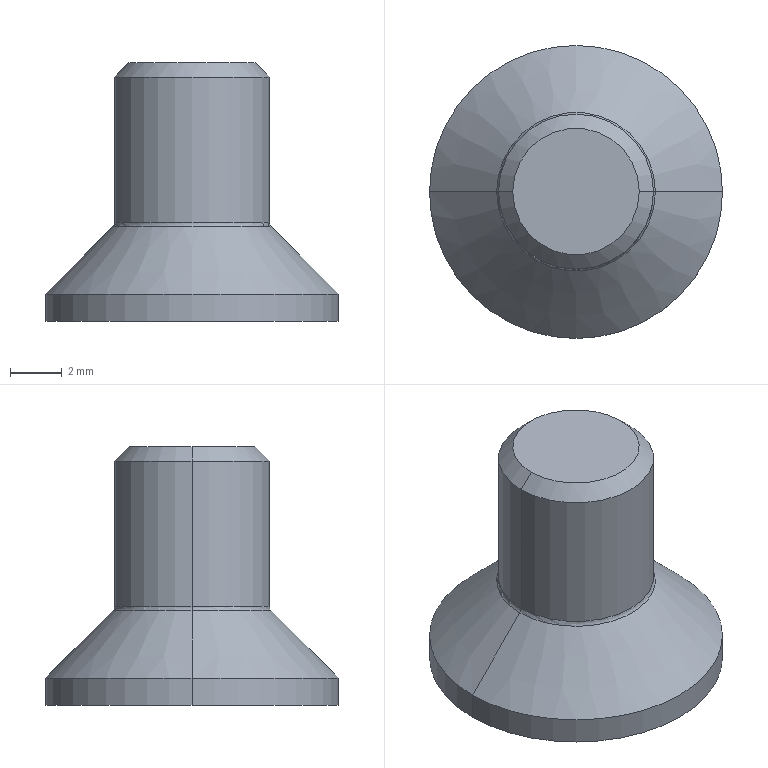Component | SolidWorks | hexagon socket countersunk head screws gb-1 | 1 solid | 26 faces | box 11.34 x 11.34 x 10 mm | volume 423 mm3 | plane 14 | cone 6 | cylinder 4 | torus 2 | commonest cylinder face diameters 11.34 x2 6 x2
build123d program:
from build123d import *

# Parameters (mm, degrees)
HEXAGONSOCKET_DEPTH = 1.1
HEADFILLET_R        = 0.25
CHAMFER_2_SIZE      = 0.55
SKETCH4_W           = 5
SKETCH4_H           = 5


with BuildPart() as part:
    # Sketch1 → Base (revolve)
    with BuildSketch(Plane.XY, mode=Mode.PRIVATE) as base_sk:
        Polygon((0, 0), (0, 6.72), (3.72, 3), (10, 3), (10, 0), align=None)
    revolve(base_sk.sketch.rotate(Axis((-0.5871, 0, 0), (1, 0, 0)), 90), axis=Axis((-0.5871, 0, 0), (1, 0, 0)))

    # Sketch2 → HexagonSocket (cut)
    with BuildSketch(Plane(origin=(0, 0, 0), x_dir=(0, 0, -1), z_dir=(1, 0, 0))):
        Polygon((2.309, 0), (1.155, 2), (-1.155, 2), (-2.309, 0), (-1.155, -2), (1.155, -2), align=None)
    extrude(amount=HEXAGONSOCKET_DEPTH, mode=Mode.SUBTRACT)

    # Sketch3 → Cut-Revolve1 (revolve, cut)
    with BuildSketch(Plane.XY, mode=Mode.PRIVATE) as cut_revolve1_sk:
        Polygon((1.1, 2), (2.255, 0), (1.1, 0), align=None)
    revolve(cut_revolve1_sk.sketch.rotate(Axis((-0.4391, 0, 0), (1, 0, 0)), 90), axis=Axis((-0.4391, 0, 0), (1, 0, 0)), mode=Mode.SUBTRACT)

    # HeadFillet
    headfillet_edges = [part.edges().sort_by_distance(p)[0] for p in [
        (3.72, 0, -3),
    ]]
    fillet(headfillet_edges, radius=HEADFILLET_R)

    # Chamfer 2
    chamfer_2_edges = [part.edges().sort_by_distance(p)[0] for p in [
        (10, 0, -3),
    ]]
    chamfer(chamfer_2_edges, length=CHAMFER_2_SIZE)

    # Sketch4 → Cut-Revolve2 (revolve, cut)
    with BuildSketch(Plane(origin=(0, 0, 0), x_dir=(1, 0, 0), z_dir=(0, 1, 0)), mode=Mode.PRIVATE) as cut_revolve2_sk:
        with Locations((0.5, 8.17)):
            Rectangle(SKETCH4_W, SKETCH4_H)
    revolve(cut_revolve2_sk.sketch.rotate(Axis((11.853, 0, 0), (-1, 0, 0)), 180), axis=Axis((11.853, 0, 0), (-1, 0, 0)), mode=Mode.SUBTRACT)


solid = part.part

# Placed as in the assembly
solid = solid.moved(Location((21.481, 88.385, 42.5), (0, -90, 0)))
STEP:
#1=CARTESIAN_POINT('',(0.8457,3.48,1.762));
#2=VERTEX_POINT('',#1);
#3=CARTESIAN_POINT('',(0.767,3.48,1.717));
#4=VERTEX_POINT('',#3);
#5=CARTESIAN_POINT('',(0.8457,3.48,1.762));
#6=DIRECTION('',(-0.866,-0.,-0.5));
#7=VECTOR('',#6,39.37);
#8=LINE('',#5,#7);
#9=EDGE_CURVE('',#2,#4,#8,.T.);
#10=ORIENTED_EDGE('',*,*,#9,.F.);
#11=CARTESIAN_POINT('',(0.9244,3.48,1.717));
#12=VERTEX_POINT('',#11);
#13=CARTESIAN_POINT('',(0.8457,3.48,1.762));
#14=DIRECTION('',(0.866,0.,-0.5));
#15=VECTOR('',#14,39.37);
#16=LINE('',#13,#15);
#17=EDGE_CURVE('',#2,#12,#16,.T.);
#18=ORIENTED_EDGE('',*,*,#17,.T.);
#19=CARTESIAN_POINT('',(0.9139,3.44,1.717));
#20=VERTEX_POINT('',#19);
#21=CARTESIAN_POINT('',(0.8457,3.48,1.717));
#22=DIRECTION('',(0.,-0.,-1.));
#23=DIRECTION('',(-1.,0.,0.));
#24=AXIS2_PLACEMENT_3D('',#21,#22,#23);
#25=CIRCLE('',#24,0.07874);
#26=EDGE_CURVE('',#12,#20,#25,.T.);
#27=ORIENTED_EDGE('',*,*,#26,.T.);
#28=CARTESIAN_POINT('',(0.8457,3.401,1.717));
#29=VERTEX_POINT('',#28);
#30=CARTESIAN_POINT('',(0.8457,3.48,1.717));
#31=DIRECTION('',(0.,-0.,-1.));
#32=DIRECTION('',(-1.,0.,0.));
#33=AXIS2_PLACEMENT_3D('',#30,#31,#32);
#34=CIRCLE('',#33,0.07874);
#35=EDGE_CURVE('',#20,#29,#34,.T.);
#36=ORIENTED_EDGE('',*,*,#35,.T.);
#37=CARTESIAN_POINT('',(0.7775,3.44,1.717));
#38=VERTEX_POINT('',#37);
#39=CARTESIAN_POINT('',(0.8457,3.48,1.717));
#40=DIRECTION('',(0.,-0.,-1.));
#41=DIRECTION('',(-1.,0.,0.));
#42=AXIS2_PLACEMENT_3D('',#39,#40,#41);
#43=CIRCLE('',#42,0.07874);
#44=EDGE_CURVE('',#29,#38,#43,.T.);
#45=ORIENTED_EDGE('',*,*,#44,.T.);
#46=CARTESIAN_POINT('',(0.8457,3.48,1.717));
#47=DIRECTION('',(0.,-0.,-1.));
#48=DIRECTION('',(-1.,0.,0.));
#49=AXIS2_PLACEMENT_3D('',#46,#47,#48);
#50=CIRCLE('',#49,0.07874);
#51=EDGE_CURVE('',#38,#4,#50,.T.);
#52=ORIENTED_EDGE('',*,*,#51,.T.);
#53=EDGE_LOOP('',(#10,#18,#27,#36,#45,#52));
#54=FACE_OUTER_BOUND('',#53,.T.);
#55=CARTESIAN_POINT('',(0.8457,3.48,-37.608));
#56=DIRECTION('',(0.,-0.,-1.));
#57=DIRECTION('',(-1.,-0.,0.));
#58=AXIS2_PLACEMENT_3D('',#55,#56,#57);
#59=CONICAL_SURFACE('',#58,68.191,1.047);
#60=ADVANCED_FACE('',(#54),#59,.F.);
#61=CARTESIAN_POINT('',(0.6225,3.48,1.673));
#62=VERTEX_POINT('',#61);
#63=CARTESIAN_POINT('',(1.069,3.48,1.673));
#64=VERTEX_POINT('',#63);
#65=CARTESIAN_POINT('',(0.8457,3.48,1.673));
#66=DIRECTION('',(0.,-0.,-1.));
#67=DIRECTION('',(1.,0.,0.));
#68=AXIS2_PLACEMENT_3D('',#65,#66,#67);
#69=CIRCLE('',#68,0.2232);
#70=EDGE_CURVE('',#62,#64,#69,.T.);
#71=ORIENTED_EDGE('',*,*,#70,.F.);
#72=CARTESIAN_POINT('',(0.6225,3.48,1.715));
#73=VERTEX_POINT('',#72);
#74=CARTESIAN_POINT('',(0.6225,3.48,2.14));
#75=DIRECTION('',(-0.,0.,1.));
#76=VECTOR('',#75,39.37);
#77=LINE('',#74,#76);
#78=EDGE_CURVE('',#62,#73,#77,.T.);
#79=ORIENTED_EDGE('',*,*,#78,.T.);
#80=CARTESIAN_POINT('',(1.069,3.48,1.715));
#81=VERTEX_POINT('',#80);
#82=CARTESIAN_POINT('',(0.8457,3.48,1.715));
#83=DIRECTION('',(-0.,0.,1.));
#84=DIRECTION('',(-1.,0.,0.));
#85=AXIS2_PLACEMENT_3D('',#82,#83,#84);
#86=CIRCLE('',#85,0.2232);
#87=EDGE_CURVE('',#81,#73,#86,.T.);
#88=ORIENTED_EDGE('',*,*,#87,.F.);
#89=CARTESIAN_POINT('',(1.069,3.48,2.14));
#90=DIRECTION('',(-0.,0.,1.));
#91=VECTOR('',#90,39.37);
#92=LINE('',#89,#91);
#93=EDGE_CURVE('',#64,#81,#92,.T.);
#94=ORIENTED_EDGE('',*,*,#93,.F.);
#95=EDGE_LOOP('',(#71,#79,#88,#94));
#96=FACE_OUTER_BOUND('',#95,.T.);
#97=CARTESIAN_POINT('',(0.8457,3.48,2.14));
#98=DIRECTION('',(-0.,0.,1.));
#99=DIRECTION('',(1.,0.,0.));
#100=AXIS2_PLACEMENT_3D('',#97,#98,#99);
#101=CYLINDRICAL_SURFACE('',#100,0.2232);
#102=ADVANCED_FACE('',(#96),#101,.T.);
#103=CARTESIAN_POINT('',(0.9422,3.48,2.067));
#104=VERTEX_POINT('',#103);
#105=CARTESIAN_POINT('',(0.7492,3.48,2.067));
#106=VERTEX_POINT('',#105);
#107=CARTESIAN_POINT('',(0.8457,3.48,2.067));
#108=DIRECTION('',(-0.,0.,1.));
#109=DIRECTION('',(-1.,0.,0.));
#110=AXIS2_PLACEMENT_3D('',#107,#108,#109);
#111=CIRCLE('',#110,0.09646);
#112=EDGE_CURVE('',#104,#106,#111,.T.);
#113=ORIENTED_EDGE('',*,*,#112,.F.);
#114=CARTESIAN_POINT('',(0.9638,3.48,2.045));
#115=VERTEX_POINT('',#114);
#116=CARTESIAN_POINT('',(0.9638,3.48,2.045));
#117=DIRECTION('',(0.7071,0.,-0.7071));
#118=VECTOR('',#117,39.37);
#119=LINE('',#116,#118);
#120=EDGE_CURVE('',#104,#115,#119,.T.);
#121=ORIENTED_EDGE('',*,*,#120,.T.);
#122=CARTESIAN_POINT('',(0.7276,3.48,2.045));
#123=VERTEX_POINT('',#122);
#124=CARTESIAN_POINT('',(0.8457,3.48,2.045));
#125=DIRECTION('',(0.,-0.,-1.));
#126=DIRECTION('',(-1.,0.,0.));
#127=AXIS2_PLACEMENT_3D('',#124,#125,#126);
#128=CIRCLE('',#127,0.1181);
#129=EDGE_CURVE('',#123,#115,#128,.T.);
#130=ORIENTED_EDGE('',*,*,#129,.F.);
#131=CARTESIAN_POINT('',(0.7276,3.48,2.045));
#132=DIRECTION('',(-0.7071,-0.,-0.7071));
#133=VECTOR('',#132,39.37);
#134=LINE('',#131,#133);
#135=EDGE_CURVE('',#106,#123,#134,.T.);
#136=ORIENTED_EDGE('',*,*,#135,.F.);
#137=EDGE_LOOP('',(#113,#121,#130,#136));
#138=FACE_OUTER_BOUND('',#137,.T.);
#139=CARTESIAN_POINT('',(0.8457,3.48,2.045));
#140=DIRECTION('',(0.,-0.,-1.));
#141=DIRECTION('',(-1.,0.,0.));
#142=AXIS2_PLACEMENT_3D('',#139,#140,#141);
#143=CONICAL_SURFACE('',#142,0.1181,0.7854);
#144=ADVANCED_FACE('',(#138),#143,.T.);
#145=CARTESIAN_POINT('',(0.9667,3.48,1.817));
#146=VERTEX_POINT('',#145);
#147=CARTESIAN_POINT('',(0.7247,3.48,1.817));
#148=VERTEX_POINT('',#147);
#149=CARTESIAN_POINT('',(0.8457,3.48,1.817));
#150=DIRECTION('',(0.,-0.,-1.));
#151=DIRECTION('',(-1.,0.,0.));
#152=AXIS2_PLACEMENT_3D('',#149,#150,#151);
#153=CIRCLE('',#152,0.121);
#154=EDGE_CURVE('',#146,#148,#153,.T.);
#155=ORIENTED_EDGE('',*,*,#154,.F.);
#156=CARTESIAN_POINT('',(0.9638,3.48,1.824));
#157=VERTEX_POINT('',#156);
#158=CARTESIAN_POINT('',(0.9736,3.48,1.824));
#159=DIRECTION('',(-0.,1.,-0.));
#160=DIRECTION('',(-1.,0.,0.));
#161=AXIS2_PLACEMENT_3D('',#158,#159,#160);
#162=CIRCLE('',#161,0.009843);
#163=EDGE_CURVE('',#146,#157,#162,.T.);
#164=ORIENTED_EDGE('',*,*,#163,.T.);
#165=CARTESIAN_POINT('',(0.7276,3.48,1.824));
#166=VERTEX_POINT('',#165);
#167=CARTESIAN_POINT('',(0.8457,3.48,1.824));
#168=DIRECTION('',(-0.,0.,1.));
#169=DIRECTION('',(-1.,0.,0.));
#170=AXIS2_PLACEMENT_3D('',#167,#168,#169);
#171=CIRCLE('',#170,0.1181);
#172=EDGE_CURVE('',#166,#157,#171,.T.);
#173=ORIENTED_EDGE('',*,*,#172,.F.);
#174=CARTESIAN_POINT('',(0.7177,3.48,1.824));
#175=DIRECTION('',(0.,-1.,0.));
#176=DIRECTION('',(0.,0.,-1.));
#177=AXIS2_PLACEMENT_3D('',#174,#175,#176);
#178=CIRCLE('',#177,0.009843);
#179=EDGE_CURVE('',#148,#166,#178,.T.);
#180=ORIENTED_EDGE('',*,*,#179,.F.);
#181=EDGE_LOOP('',(#155,#164,#173,#180));
#182=FACE_OUTER_BOUND('',#181,.T.);
#183=CARTESIAN_POINT('',(0.8457,3.48,1.824));
#184=DIRECTION('',(0.,-0.,-1.));
#185=DIRECTION('',(-1.,-0.,-0.));
#186=AXIS2_PLACEMENT_3D('',#183,#184,#185);
#187=TOROIDAL_SURFACE('',#186,0.128,0.009843);
#188=ADVANCED_FACE('',(#182),#187,.F.);
#189=CARTESIAN_POINT('',(0.8457,3.48,1.817));
#190=DIRECTION('',(0.,-0.,-1.));
#191=DIRECTION('',(-1.,0.,0.));
#192=AXIS2_PLACEMENT_3D('',#189,#190,#191);
#193=CIRCLE('',#192,0.121);
#194=EDGE_CURVE('',#148,#146,#193,.T.);
#195=ORIENTED_EDGE('',*,*,#194,.T.);
#196=CARTESIAN_POINT('',(0.9638,3.48,1.82));
#197=DIRECTION('',(0.7071,0.,-0.7071));
#198=VECTOR('',#197,39.37);
#199=LINE('',#196,#198);
#200=EDGE_CURVE('',#146,#81,#199,.T.);
#201=ORIENTED_EDGE('',*,*,#200,.T.);
#202=ORIENTED_EDGE('',*,*,#87,.T.);
#203=CARTESIAN_POINT('',(0.7276,3.48,1.82));
#204=DIRECTION('',(-0.7071,-0.,-0.7071));
#205=VECTOR('',#204,39.37);
#206=LINE('',#203,#205);
#207=EDGE_CURVE('',#148,#73,#206,.T.);
#208=ORIENTED_EDGE('',*,*,#207,.F.);
#209=EDGE_LOOP('',(#195,#201,#202,#208));
#210=FACE_OUTER_BOUND('',#209,.T.);
#211=CARTESIAN_POINT('',(0.8457,3.48,1.82));
#212=DIRECTION('',(0.,-0.,-1.));
#213=DIRECTION('',(-1.,0.,0.));
#214=AXIS2_PLACEMENT_3D('',#211,#212,#213);
#215=CONICAL_SURFACE('',#214,0.1181,0.7854);
#216=ADVANCED_FACE('',(#210),#215,.T.);
#217=ORIENTED_EDGE('',*,*,#129,.T.);
#218=CARTESIAN_POINT('',(0.9638,3.48,1.65));
#219=DIRECTION('',(0.,-0.,-1.));
#220=VECTOR('',#219,39.37);
#221=LINE('',#218,#220);
#222=EDGE_CURVE('',#115,#157,#221,.T.);
#223=ORIENTED_EDGE('',*,*,#222,.T.);
#224=CARTESIAN_POINT('',(0.8457,3.48,1.824));
#225=DIRECTION('',(-0.,0.,1.));
#226=DIRECTION('',(-1.,0.,0.));
#227=AXIS2_PLACEMENT_3D('',#224,#225,#226);
#228=CIRCLE('',#227,0.1181);
#229=EDGE_CURVE('',#157,#166,#228,.T.);
#230=ORIENTED_EDGE('',*,*,#229,.T.);
#231=CARTESIAN_POINT('',(0.7276,3.48,1.65));
#232=DIRECTION('',(0.,-0.,-1.));
#233=VECTOR('',#232,39.37);
#234=LINE('',#231,#233);
#235=EDGE_CURVE('',#123,#166,#234,.T.);
#236=ORIENTED_EDGE('',*,*,#235,.F.);
#237=EDGE_LOOP('',(#217,#223,#230,#236));
#238=FACE_OUTER_BOUND('',#237,.T.);
#239=CARTESIAN_POINT('',(0.8457,3.48,1.65));
#240=DIRECTION('',(0.,-0.,-1.));
#241=DIRECTION('',(-1.,0.,0.));
#242=AXIS2_PLACEMENT_3D('',#239,#240,#241);
#243=CYLINDRICAL_SURFACE('',#242,0.1181);
#244=ADVANCED_FACE('',(#238),#243,.T.);
#245=CARTESIAN_POINT('',(0.8457,3.48,2.067));
#246=DIRECTION('',(-0.,0.,1.));
#247=DIRECTION('',(-1.,0.,0.));
#248=AXIS2_PLACEMENT_3D('',#245,#246,#247);
#249=CIRCLE('',#248,0.09646);
#250=EDGE_CURVE('',#106,#104,#249,.T.);
#251=ORIENTED_EDGE('',*,*,#250,.T.);
#252=ORIENTED_EDGE('',*,*,#112,.T.);
#253=EDGE_LOOP('',(#251,#252));
#254=FACE_OUTER_BOUND('',#253,.T.);
#255=CARTESIAN_POINT('',(0.8457,3.598,2.067));
#256=DIRECTION('',(0.,-0.,-1.));
#257=DIRECTION('',(-1.,-0.,-0.));
#258=AXIS2_PLACEMENT_3D('',#255,#256,#257);
#259=PLANE('',#258);
#260=ADVANCED_FACE('',(#254),#259,.F.);
#261=ORIENTED_EDGE('',*,*,#222,.F.);
#262=CARTESIAN_POINT('',(0.8457,3.48,2.045));
#263=DIRECTION('',(0.,-0.,-1.));
#264=DIRECTION('',(-1.,0.,0.));
#265=AXIS2_PLACEMENT_3D('',#262,#263,#264);
#266=CIRCLE('',#265,0.1181);
#267=EDGE_CURVE('',#115,#123,#266,.T.);
#268=ORIENTED_EDGE('',*,*,#267,.T.);
#269=ORIENTED_EDGE('',*,*,#235,.T.);
#270=ORIENTED_EDGE('',*,*,#172,.T.);
#271=EDGE_LOOP('',(#261,#268,#269,#270));
#272=FACE_OUTER_BOUND('',#271,.T.);
#273=CARTESIAN_POINT('',(0.8457,3.48,1.65));
#274=DIRECTION('',(0.,-0.,-1.));
#275=DIRECTION('',(-1.,0.,0.));
#276=AXIS2_PLACEMENT_3D('',#273,#274,#275);
#277=CYLINDRICAL_SURFACE('',#276,0.1181);
#278=ADVANCED_FACE('',(#272),#277,.T.);
#279=ORIENTED_EDGE('',*,*,#200,.F.);
#280=ORIENTED_EDGE('',*,*,#154,.T.);
#281=ORIENTED_EDGE('',*,*,#207,.T.);
#282=CARTESIAN_POINT('',(0.8457,3.48,1.715));
#283=DIRECTION('',(-0.,0.,1.));
#284=DIRECTION('',(-1.,0.,0.));
#285=AXIS2_PLACEMENT_3D('',#282,#283,#284);
#286=CIRCLE('',#285,0.2232);
#287=EDGE_CURVE('',#73,#81,#286,.T.);
#288=ORIENTED_EDGE('',*,*,#287,.T.);
#289=EDGE_LOOP('',(#279,#280,#281,#288));
#290=FACE_OUTER_BOUND('',#289,.T.);
#291=CARTESIAN_POINT('',(0.8457,3.48,1.82));
#292=DIRECTION('',(0.,-0.,-1.));
#293=DIRECTION('',(-1.,0.,0.));
#294=AXIS2_PLACEMENT_3D('',#291,#292,#293);
#295=CONICAL_SURFACE('',#294,0.1181,0.7854);
#296=ADVANCED_FACE('',(#290),#295,.T.);
#297=ORIENTED_EDGE('',*,*,#163,.F.);
#298=ORIENTED_EDGE('',*,*,#194,.F.);
#299=ORIENTED_EDGE('',*,*,#179,.T.);
#300=ORIENTED_EDGE('',*,*,#229,.F.);
#301=EDGE_LOOP('',(#297,#298,#299,#300));
#302=FACE_OUTER_BOUND('',#301,.T.);
#303=CARTESIAN_POINT('',(0.8457,3.48,1.824));
#304=DIRECTION('',(0.,-0.,-1.));
#305=DIRECTION('',(-1.,-0.,-0.));
#306=AXIS2_PLACEMENT_3D('',#303,#304,#305);
#307=TOROIDAL_SURFACE('',#306,0.128,0.009843);
#308=ADVANCED_FACE('',(#302),#307,.F.);
#309=ORIENTED_EDGE('',*,*,#120,.F.);
#310=ORIENTED_EDGE('',*,*,#250,.F.);
#311=ORIENTED_EDGE('',*,*,#135,.T.);
#312=ORIENTED_EDGE('',*,*,#267,.F.);
#313=EDGE_LOOP('',(#309,#310,#311,#312));
#314=FACE_OUTER_BOUND('',#313,.T.);
#315=CARTESIAN_POINT('',(0.8457,3.48,2.045));
#316=DIRECTION('',(0.,-0.,-1.));
#317=DIRECTION('',(-1.,0.,0.));
#318=AXIS2_PLACEMENT_3D('',#315,#316,#317);
#319=CONICAL_SURFACE('',#318,0.1181,0.7854);
#320=ADVANCED_FACE('',(#314),#319,.T.);
#321=ORIENTED_EDGE('',*,*,#78,.F.);
#322=CARTESIAN_POINT('',(0.8457,3.48,1.673));
#323=DIRECTION('',(0.,-0.,-1.));
#324=DIRECTION('',(1.,0.,0.));
#325=AXIS2_PLACEMENT_3D('',#322,#323,#324);
#326=CIRCLE('',#325,0.2232);
#327=EDGE_CURVE('',#64,#62,#326,.T.);
#328=ORIENTED_EDGE('',*,*,#327,.F.);
#329=ORIENTED_EDGE('',*,*,#93,.T.);
#330=ORIENTED_EDGE('',*,*,#287,.F.);
#331=EDGE_LOOP('',(#321,#328,#329,#330));
#332=FACE_OUTER_BOUND('',#331,.T.);
#333=CARTESIAN_POINT('',(0.8457,3.48,2.14));
#334=DIRECTION('',(-0.,0.,1.));
#335=DIRECTION('',(1.,0.,0.));
#336=AXIS2_PLACEMENT_3D('',#333,#334,#335);
#337=CYLINDRICAL_SURFACE('',#336,0.2232);
#338=ADVANCED_FACE('',(#332),#337,.T.);
#339=ORIENTED_EDGE('',*,*,#17,.F.);
#340=ORIENTED_EDGE('',*,*,#9,.T.);
#341=CARTESIAN_POINT('',(0.7775,3.519,1.717));
#342=VERTEX_POINT('',#341);
#343=CARTESIAN_POINT('',(0.8457,3.48,1.717));
#344=DIRECTION('',(0.,-0.,-1.));
#345=DIRECTION('',(-1.,0.,0.));
#346=AXIS2_PLACEMENT_3D('',#343,#344,#345);
#347=CIRCLE('',#346,0.07874);
#348=EDGE_CURVE('',#4,#342,#347,.T.);
#349=ORIENTED_EDGE('',*,*,#348,.T.);
#350=CARTESIAN_POINT('',(0.8457,3.558,1.717));
#351=VERTEX_POINT('',#350);
#352=CARTESIAN_POINT('',(0.8457,3.48,1.717));
#353=DIRECTION('',(0.,-0.,-1.));
#354=DIRECTION('',(-1.,0.,0.));
#355=AXIS2_PLACEMENT_3D('',#352,#353,#354);
#356=CIRCLE('',#355,0.07874);
#357=EDGE_CURVE('',#342,#351,#356,.T.);
#358=ORIENTED_EDGE('',*,*,#357,.T.);
#359=CARTESIAN_POINT('',(0.9139,3.519,1.717));
#360=VERTEX_POINT('',#359);
#361=CARTESIAN_POINT('',(0.8457,3.48,1.717));
#362=DIRECTION('',(0.,-0.,-1.));
#363=DIRECTION('',(-1.,0.,0.));
#364=AXIS2_PLACEMENT_3D('',#361,#362,#363);
#365=CIRCLE('',#364,0.07874);
#366=EDGE_CURVE('',#351,#360,#365,.T.);
#367=ORIENTED_EDGE('',*,*,#366,.T.);
#368=CARTESIAN_POINT('',(0.8457,3.48,1.717));
#369=DIRECTION('',(0.,-0.,-1.));
#370=DIRECTION('',(-1.,0.,0.));
#371=AXIS2_PLACEMENT_3D('',#368,#369,#370);
#372=CIRCLE('',#371,0.07874);
#373=EDGE_CURVE('',#360,#12,#372,.T.);
#374=ORIENTED_EDGE('',*,*,#373,.T.);
#375=EDGE_LOOP('',(#339,#340,#349,#358,#367,#374));
#376=FACE_OUTER_BOUND('',#375,.T.);
#377=CARTESIAN_POINT('',(0.8457,3.48,-37.608));
#378=DIRECTION('',(0.,-0.,-1.));
#379=DIRECTION('',(-1.,-0.,0.));
#380=AXIS2_PLACEMENT_3D('',#377,#378,#379);
#381=CONICAL_SURFACE('',#380,68.191,1.047);
#382=ADVANCED_FACE('',(#376),#381,.F.);
#383=ORIENTED_EDGE('',*,*,#44,.F.);
#384=CARTESIAN_POINT('',(0.8002,3.401,1.717));
#385=VERTEX_POINT('',#384);
#386=CARTESIAN_POINT('',(0.8002,3.401,1.717));
#387=DIRECTION('',(1.,0.,0.));
#388=VECTOR('',#387,39.37);
#389=LINE('',#386,#388);
#390=EDGE_CURVE('',#385,#29,#389,.T.);
#391=ORIENTED_EDGE('',*,*,#390,.F.);
#392=CARTESIAN_POINT('',(0.7548,3.48,1.717));
#393=DIRECTION('',(0.5,-0.866,0.));
#394=VECTOR('',#393,39.37);
#395=LINE('',#392,#394);
#396=EDGE_CURVE('',#38,#385,#395,.T.);
#397=ORIENTED_EDGE('',*,*,#396,.F.);
#398=EDGE_LOOP('',(#383,#391,#397));
#399=FACE_OUTER_BOUND('',#398,.T.);
#400=CARTESIAN_POINT('',(0.9366,3.48,1.717));
#401=DIRECTION('',(-0.,0.,1.));
#402=DIRECTION('',(1.,0.,0.));
#403=AXIS2_PLACEMENT_3D('',#400,#401,#402);
#404=PLANE('',#403);
#405=ADVANCED_FACE('',(#399),#404,.F.);
#406=ORIENTED_EDGE('',*,*,#51,.F.);
#407=CARTESIAN_POINT('',(0.7548,3.48,1.717));
#408=VERTEX_POINT('',#407);
#409=CARTESIAN_POINT('',(0.7548,3.48,1.717));
#410=DIRECTION('',(0.5,-0.866,0.));
#411=VECTOR('',#410,39.37);
#412=LINE('',#409,#411);
#413=EDGE_CURVE('',#408,#38,#412,.T.);
#414=ORIENTED_EDGE('',*,*,#413,.F.);
#415=CARTESIAN_POINT('',(0.8002,3.558,1.717));
#416=DIRECTION('',(-0.5,-0.866,0.));
#417=VECTOR('',#416,39.37);
#418=LINE('',#415,#417);
#419=EDGE_CURVE('',#342,#408,#418,.T.);
#420=ORIENTED_EDGE('',*,*,#419,.F.);
#421=ORIENTED_EDGE('',*,*,#348,.F.);
#422=EDGE_LOOP('',(#406,#414,#420,#421));
#423=FACE_OUTER_BOUND('',#422,.T.);
#424=CARTESIAN_POINT('',(0.9366,3.48,1.717));
#425=DIRECTION('',(-0.,0.,1.));
#426=DIRECTION('',(1.,0.,0.));
#427=AXIS2_PLACEMENT_3D('',#424,#425,#426);
#428=PLANE('',#427);
#429=ADVANCED_FACE('',(#423),#428,.F.);
#430=ORIENTED_EDGE('',*,*,#357,.F.);
#431=CARTESIAN_POINT('',(0.8002,3.558,1.717));
#432=VERTEX_POINT('',#431);
#433=CARTESIAN_POINT('',(0.8002,3.558,1.717));
#434=DIRECTION('',(-0.5,-0.866,0.));
#435=VECTOR('',#434,39.37);
#436=LINE('',#433,#435);
#437=EDGE_CURVE('',#432,#342,#436,.T.);
#438=ORIENTED_EDGE('',*,*,#437,.F.);
#439=CARTESIAN_POINT('',(0.8912,3.558,1.717));
#440=DIRECTION('',(-1.,-0.,-0.));
#441=VECTOR('',#440,39.37);
#442=LINE('',#439,#441);
#443=EDGE_CURVE('',#351,#432,#442,.T.);
#444=ORIENTED_EDGE('',*,*,#443,.F.);
#445=EDGE_LOOP('',(#430,#438,#444));
#446=FACE_OUTER_BOUND('',#445,.T.);
#447=CARTESIAN_POINT('',(0.9366,3.48,1.717));
#448=DIRECTION('',(-0.,0.,1.));
#449=DIRECTION('',(1.,0.,0.));
#450=AXIS2_PLACEMENT_3D('',#447,#448,#449);
#451=PLANE('',#450);
#452=ADVANCED_FACE('',(#446),#451,.F.);
#453=ORIENTED_EDGE('',*,*,#366,.F.);
#454=CARTESIAN_POINT('',(0.8912,3.558,1.717));
#455=VERTEX_POINT('',#454);
#456=CARTESIAN_POINT('',(0.8912,3.558,1.717));
#457=DIRECTION('',(-1.,-0.,-0.));
#458=VECTOR('',#457,39.37);
#459=LINE('',#456,#458);
#460=EDGE_CURVE('',#455,#351,#459,.T.);
#461=ORIENTED_EDGE('',*,*,#460,.F.);
#462=CARTESIAN_POINT('',(0.9366,3.48,1.717));
#463=DIRECTION('',(-0.5,0.866,-0.));
#464=VECTOR('',#463,39.37);
#465=LINE('',#462,#464);
#466=EDGE_CURVE('',#360,#455,#465,.T.);
#467=ORIENTED_EDGE('',*,*,#466,.F.);
#468=EDGE_LOOP('',(#453,#461,#467));
#469=FACE_OUTER_BOUND('',#468,.T.);
#470=CARTESIAN_POINT('',(0.9366,3.48,1.717));
#471=DIRECTION('',(-0.,0.,1.));
#472=DIRECTION('',(1.,0.,0.));
#473=AXIS2_PLACEMENT_3D('',#470,#471,#472);
#474=PLANE('',#473);
#475=ADVANCED_FACE('',(#469),#474,.F.);
#476=ORIENTED_EDGE('',*,*,#373,.F.);
#477=CARTESIAN_POINT('',(0.9366,3.48,1.717));
#478=VERTEX_POINT('',#477);
#479=CARTESIAN_POINT('',(0.9366,3.48,1.717));
#480=DIRECTION('',(-0.5,0.866,-0.));
#481=VECTOR('',#480,39.37);
#482=LINE('',#479,#481);
#483=EDGE_CURVE('',#478,#360,#482,.T.);
#484=ORIENTED_EDGE('',*,*,#483,.F.);
#485=CARTESIAN_POINT('',(0.8912,3.401,1.717));
#486=DIRECTION('',(0.5,0.866,-0.));
#487=VECTOR('',#486,39.37);
#488=LINE('',#485,#487);
#489=EDGE_CURVE('',#20,#478,#488,.T.);
#490=ORIENTED_EDGE('',*,*,#489,.F.);
#491=ORIENTED_EDGE('',*,*,#26,.F.);
#492=EDGE_LOOP('',(#476,#484,#490,#491));
#493=FACE_OUTER_BOUND('',#492,.T.);
#494=CARTESIAN_POINT('',(0.9366,3.48,1.717));
#495=DIRECTION('',(-0.,0.,1.));
#496=DIRECTION('',(1.,0.,0.));
#497=AXIS2_PLACEMENT_3D('',#494,#495,#496);
#498=PLANE('',#497);
#499=ADVANCED_FACE('',(#493),#498,.F.);
#500=ORIENTED_EDGE('',*,*,#35,.F.);
#501=CARTESIAN_POINT('',(0.8912,3.401,1.717));
#502=VERTEX_POINT('',#501);
#503=CARTESIAN_POINT('',(0.8912,3.401,1.717));
#504=DIRECTION('',(0.5,0.866,-0.));
#505=VECTOR('',#504,39.37);
#506=LINE('',#503,#505);
#507=EDGE_CURVE('',#502,#20,#506,.T.);
#508=ORIENTED_EDGE('',*,*,#507,.F.);
#509=CARTESIAN_POINT('',(0.8002,3.401,1.717));
#510=DIRECTION('',(1.,0.,0.));
#511=VECTOR('',#510,39.37);
#512=LINE('',#509,#511);
#513=EDGE_CURVE('',#29,#502,#512,.T.);
#514=ORIENTED_EDGE('',*,*,#513,.F.);
#515=EDGE_LOOP('',(#500,#508,#514));
#516=FACE_OUTER_BOUND('',#515,.T.);
#517=CARTESIAN_POINT('',(0.9366,3.48,1.717));
#518=DIRECTION('',(-0.,0.,1.));
#519=DIRECTION('',(1.,0.,0.));
#520=AXIS2_PLACEMENT_3D('',#517,#518,#519);
#521=PLANE('',#520);
#522=ADVANCED_FACE('',(#516),#521,.F.);
#523=CARTESIAN_POINT('',(0.8002,3.401,1.673));
#524=VERTEX_POINT('',#523);
#525=CARTESIAN_POINT('',(0.8912,3.401,1.673));
#526=VERTEX_POINT('',#525);
#527=CARTESIAN_POINT('',(0.8002,3.401,1.673));
#528=DIRECTION('',(1.,0.,0.));
#529=VECTOR('',#528,39.37);
#530=LINE('',#527,#529);
#531=EDGE_CURVE('',#524,#526,#530,.T.);
#532=ORIENTED_EDGE('',*,*,#531,.F.);
#533=CARTESIAN_POINT('',(0.8002,3.401,1.717));
#534=DIRECTION('',(0.,-0.,-1.));
#535=VECTOR('',#534,39.37);
#536=LINE('',#533,#535);
#537=EDGE_CURVE('',#385,#524,#536,.T.);
#538=ORIENTED_EDGE('',*,*,#537,.F.);
#539=ORIENTED_EDGE('',*,*,#390,.T.);
#540=ORIENTED_EDGE('',*,*,#513,.T.);
#541=CARTESIAN_POINT('',(0.8912,3.401,1.717));
#542=DIRECTION('',(0.,-0.,-1.));
#543=VECTOR('',#542,39.37);
#544=LINE('',#541,#543);
#545=EDGE_CURVE('',#502,#526,#544,.T.);
#546=ORIENTED_EDGE('',*,*,#545,.T.);
#547=EDGE_LOOP('',(#532,#538,#539,#540,#546));
#548=FACE_OUTER_BOUND('',#547,.T.);
#549=CARTESIAN_POINT('',(0.8002,3.401,1.717));
#550=DIRECTION('',(-0.,1.,-0.));
#551=DIRECTION('',(-1.,-0.,-0.));
#552=AXIS2_PLACEMENT_3D('',#549,#550,#551);
#553=PLANE('',#552);
#554=ADVANCED_FACE('',(#548),#553,.T.);
#555=CARTESIAN_POINT('',(0.7548,3.48,1.673));
#556=VERTEX_POINT('',#555);
#557=CARTESIAN_POINT('',(0.7548,3.48,1.673));
#558=DIRECTION('',(0.5,-0.866,0.));
#559=VECTOR('',#558,39.37);
#560=LINE('',#557,#559);
#561=EDGE_CURVE('',#556,#524,#560,.T.);
#562=ORIENTED_EDGE('',*,*,#561,.F.);
#563=CARTESIAN_POINT('',(0.7548,3.48,1.717));
#564=DIRECTION('',(0.,-0.,-1.));
#565=VECTOR('',#564,39.37);
#566=LINE('',#563,#565);
#567=EDGE_CURVE('',#408,#556,#566,.T.);
#568=ORIENTED_EDGE('',*,*,#567,.F.);
#569=ORIENTED_EDGE('',*,*,#413,.T.);
#570=ORIENTED_EDGE('',*,*,#396,.T.);
#571=ORIENTED_EDGE('',*,*,#537,.T.);
#572=EDGE_LOOP('',(#562,#568,#569,#570,#571));
#573=FACE_OUTER_BOUND('',#572,.T.);
#574=CARTESIAN_POINT('',(0.7548,3.48,1.717));
#575=DIRECTION('',(0.866,0.5,0.));
#576=DIRECTION('',(-0.5,0.866,-0.));
#577=AXIS2_PLACEMENT_3D('',#574,#575,#576);
#578=PLANE('',#577);
#579=ADVANCED_FACE('',(#573),#578,.T.);
#580=CARTESIAN_POINT('',(0.8002,3.558,1.673));
#581=VERTEX_POINT('',#580);
#582=CARTESIAN_POINT('',(0.8002,3.558,1.673));
#583=DIRECTION('',(-0.5,-0.866,0.));
#584=VECTOR('',#583,39.37);
#585=LINE('',#582,#584);
#586=EDGE_CURVE('',#581,#556,#585,.T.);
#587=ORIENTED_EDGE('',*,*,#586,.F.);
#588=CARTESIAN_POINT('',(0.8002,3.558,1.717));
#589=DIRECTION('',(0.,-0.,-1.));
#590=VECTOR('',#589,39.37);
#591=LINE('',#588,#590);
#592=EDGE_CURVE('',#432,#581,#591,.T.);
#593=ORIENTED_EDGE('',*,*,#592,.F.);
#594=ORIENTED_EDGE('',*,*,#437,.T.);
#595=ORIENTED_EDGE('',*,*,#419,.T.);
#596=ORIENTED_EDGE('',*,*,#567,.T.);
#597=EDGE_LOOP('',(#587,#593,#594,#595,#596));
#598=FACE_OUTER_BOUND('',#597,.T.);
#599=CARTESIAN_POINT('',(0.8002,3.558,1.717));
#600=DIRECTION('',(0.866,-0.5,0.));
#601=DIRECTION('',(0.5,0.866,-0.));
#602=AXIS2_PLACEMENT_3D('',#599,#600,#601);
#603=PLANE('',#602);
#604=ADVANCED_FACE('',(#598),#603,.T.);
#605=CARTESIAN_POINT('',(0.8912,3.558,1.673));
#606=VERTEX_POINT('',#605);
#607=CARTESIAN_POINT('',(0.8912,3.558,1.673));
#608=DIRECTION('',(-1.,-0.,-0.));
#609=VECTOR('',#608,39.37);
#610=LINE('',#607,#609);
#611=EDGE_CURVE('',#606,#581,#610,.T.);
#612=ORIENTED_EDGE('',*,*,#611,.F.);
#613=CARTESIAN_POINT('',(0.8912,3.558,1.717));
#614=DIRECTION('',(0.,-0.,-1.));
#615=VECTOR('',#614,39.37);
#616=LINE('',#613,#615);
#617=EDGE_CURVE('',#455,#606,#616,.T.);
#618=ORIENTED_EDGE('',*,*,#617,.F.);
#619=ORIENTED_EDGE('',*,*,#460,.T.);
#620=ORIENTED_EDGE('',*,*,#443,.T.);
#621=ORIENTED_EDGE('',*,*,#592,.T.);
#622=EDGE_LOOP('',(#612,#618,#619,#620,#621));
#623=FACE_OUTER_BOUND('',#622,.T.);
#624=CARTESIAN_POINT('',(0.8912,3.558,1.717));
#625=DIRECTION('',(0.,-1.,0.));
#626=DIRECTION('',(1.,0.,0.));
#627=AXIS2_PLACEMENT_3D('',#624,#625,#626);
#628=PLANE('',#627);
#629=ADVANCED_FACE('',(#623),#628,.T.);
#630=CARTESIAN_POINT('',(0.9366,3.48,1.673));
#631=VERTEX_POINT('',#630);
#632=CARTESIAN_POINT('',(0.9366,3.48,1.673));
#633=DIRECTION('',(-0.5,0.866,-0.));
#634=VECTOR('',#633,39.37);
#635=LINE('',#632,#634);
#636=EDGE_CURVE('',#631,#606,#635,.T.);
#637=ORIENTED_EDGE('',*,*,#636,.F.);
#638=CARTESIAN_POINT('',(0.9366,3.48,1.717));
#639=DIRECTION('',(0.,-0.,-1.));
#640=VECTOR('',#639,39.37);
#641=LINE('',#638,#640);
#642=EDGE_CURVE('',#478,#631,#641,.T.);
#643=ORIENTED_EDGE('',*,*,#642,.F.);
#644=ORIENTED_EDGE('',*,*,#483,.T.);
#645=ORIENTED_EDGE('',*,*,#466,.T.);
#646=ORIENTED_EDGE('',*,*,#617,.T.);
#647=EDGE_LOOP('',(#637,#643,#644,#645,#646));
#648=FACE_OUTER_BOUND('',#647,.T.);
#649=CARTESIAN_POINT('',(0.9366,3.48,1.717));
#650=DIRECTION('',(-0.866,-0.5,-0.));
#651=DIRECTION('',(0.5,-0.866,0.));
#652=AXIS2_PLACEMENT_3D('',#649,#650,#651);
#653=PLANE('',#652);
#654=ADVANCED_FACE('',(#648),#653,.T.);
#655=CARTESIAN_POINT('',(0.8912,3.401,1.673));
#656=DIRECTION('',(0.5,0.866,-0.));
#657=VECTOR('',#656,39.37);
#658=LINE('',#655,#657);
#659=EDGE_CURVE('',#526,#631,#658,.T.);
#660=ORIENTED_EDGE('',*,*,#659,.F.);
#661=ORIENTED_EDGE('',*,*,#545,.F.);
#662=ORIENTED_EDGE('',*,*,#507,.T.);
#663=ORIENTED_EDGE('',*,*,#489,.T.);
#664=ORIENTED_EDGE('',*,*,#642,.T.);
#665=EDGE_LOOP('',(#660,#661,#662,#663,#664));
#666=FACE_OUTER_BOUND('',#665,.T.);
#667=CARTESIAN_POINT('',(0.8912,3.401,1.717));
#668=DIRECTION('',(-0.866,0.5,-0.));
#669=DIRECTION('',(-0.5,-0.866,0.));
#670=AXIS2_PLACEMENT_3D('',#667,#668,#669);
#671=PLANE('',#670);
#672=ADVANCED_FACE('',(#666),#671,.T.);
#673=ORIENTED_EDGE('',*,*,#327,.T.);
#674=ORIENTED_EDGE('',*,*,#70,.T.);
#675=EDGE_LOOP('',(#673,#674));
#676=FACE_OUTER_BOUND('',#675,.T.);
#677=ORIENTED_EDGE('',*,*,#659,.T.);
#678=ORIENTED_EDGE('',*,*,#636,.T.);
#679=ORIENTED_EDGE('',*,*,#611,.T.);
#680=ORIENTED_EDGE('',*,*,#586,.T.);
#681=ORIENTED_EDGE('',*,*,#561,.T.);
#682=ORIENTED_EDGE('',*,*,#531,.T.);
#683=EDGE_LOOP('',(#677,#678,#679,#680,#681,#682));
#684=FACE_BOUND('',#683,.T.);
#685=CARTESIAN_POINT('',(0.8457,3.48,1.673));
#686=DIRECTION('',(-0.,0.,1.));
#687=DIRECTION('',(1.,0.,0.));
#688=AXIS2_PLACEMENT_3D('',#685,#686,#687);
#689=PLANE('',#688);
#690=ADVANCED_FACE('',(#676,#684),#689,.F.);
#691=CLOSED_SHELL('',(#60,#102,#144,#188,#216,#244,#260,#278,#296,#308,#320,#338,#382,#405,#429,#452,#475,#499,#522,#554,#579,#604,#629,#654,#672,#690));
#692=MANIFOLD_SOLID_BREP('',#691);
#693=CARTESIAN_POINT('',(0.,0.,0.));
#694=DIRECTION('',(0.,0.,1.));
#695=DIRECTION('',(1.,0.,0.));
#696=AXIS2_PLACEMENT_3D('',#693,#694,#695);
#697=(LENGTH_UNIT()NAMED_UNIT(*)SI_UNIT($,.METRE.));
#698=LENGTH_MEASURE_WITH_UNIT(LENGTH_MEASURE(0.0254),#697);
#699=DIMENSIONAL_EXPONENTS(1.,0.,0.,0.,0.,0.,0.);
#700=(CONVERSION_BASED_UNIT('',#698)LENGTH_UNIT()NAMED_UNIT(#699));
#701=UNCERTAINTY_MEASURE_WITH_UNIT(LENGTH_MEASURE(0.00001),#700,'','');
#702=(NAMED_UNIT(*)PLANE_ANGLE_UNIT()SI_UNIT($,.RADIAN.));
#703=(NAMED_UNIT(*)SI_UNIT($,.STERADIAN.)SOLID_ANGLE_UNIT());
#704=(GEOMETRIC_REPRESENTATION_CONTEXT(3)GLOBAL_UNCERTAINTY_ASSIGNED_CONTEXT((#701))GLOBAL_UNIT_ASSIGNED_CONTEXT((#700,#702,#703))REPRESENTATION_CONTEXT('',''));
#705=ADVANCED_BREP_SHAPE_REPRESENTATION('',(#692,#696),#704);
#706=COLOUR_RGB('',0.7922,0.8196,0.9333);
#707=FILL_AREA_STYLE_COLOUR('',#706);
#708=FILL_AREA_STYLE('',(#707));
#709=SURFACE_STYLE_FILL_AREA(#708);
#710=SURFACE_SIDE_STYLE('',(#709));
#711=SURFACE_STYLE_USAGE(.BOTH.,#710);
#712=PRESENTATION_STYLE_ASSIGNMENT((#711));
#713=STYLED_ITEM('',(#712),#692);
#714=PRESENTATION_LAYER_ASSIGNMENT('','',(#713));
#715=(LENGTH_UNIT()NAMED_UNIT(*)SI_UNIT($,.METRE.));
#716=LENGTH_MEASURE_WITH_UNIT(LENGTH_MEASURE(0.0254),#715);
#717=DIMENSIONAL_EXPONENTS(1.,0.,0.,0.,0.,0.,0.);
#718=(CONVERSION_BASED_UNIT('',#716)LENGTH_UNIT()NAMED_UNIT(#717));
#719=UNCERTAINTY_MEASURE_WITH_UNIT(LENGTH_MEASURE(0.00001),#718,'','');
#720=(NAMED_UNIT(*)PLANE_ANGLE_UNIT()SI_UNIT($,.RADIAN.));
#721=(NAMED_UNIT(*)SI_UNIT($,.STERADIAN.)SOLID_ANGLE_UNIT());
#722=(GEOMETRIC_REPRESENTATION_CONTEXT(3)GLOBAL_UNCERTAINTY_ASSIGNED_CONTEXT((#719))GLOBAL_UNIT_ASSIGNED_CONTEXT((#718,#720,#721))REPRESENTATION_CONTEXT('',''));
#723=MECHANICAL_DESIGN_GEOMETRIC_PRESENTATION_REPRESENTATION('',(#713),#722);